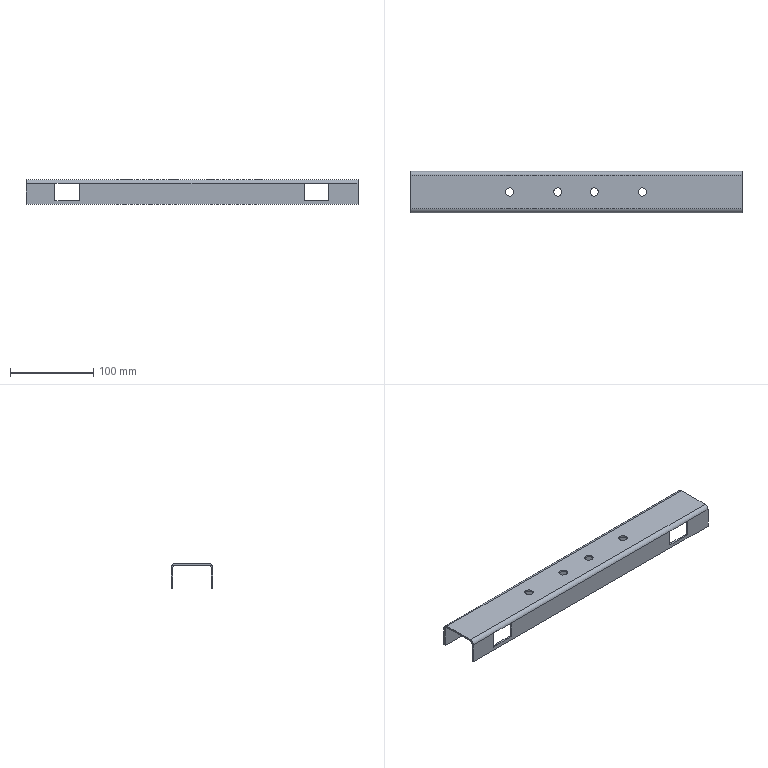Component | SolidWorks | 50x30x2ColdBentEqualAngleSteel400-1 | 1 solid | 52 faces | box 400 x 50 x 30 mm | volume 76567 mm3 | plane 34 | cylinder 18 | commonest cylinder face diameters 10 x10 6 x8
build123d program:
from build123d import *

# Parameters (mm, degrees)
BOSS_EXTRUDE1_DEPTH     = 400
SKETCH3_R               = 5
CUT_EXTRUDE1_2_DEPTH    = 65
SKETCH4_R               = 5
CUT_EXTRUDE2_DEPTH      = 65
CUT_EXTRUDE3_DEPTH      = 67
SKETCH6_W               = 30
SKETCH6_H               = 20
CUT_EXTRUDE4_DEPTH      = 67
FILLET1_R               = 3
CUT_EXTRUDE1_DEPTH      = 405.228
CUT_EXTRUDE1_DEPTH_BACK = 405.228
SKETCH1_W               = 5.72
SKETCH1_H               = 21


with BuildPart() as part:
    # Sketch1_2 → Boss-Extrude1 (new body)
    with BuildSketch(Plane(origin=(0, 0, 0), x_dir=(0, 0, -1), z_dir=(1, 0, 0))):
        with BuildLine():
            Line((0, 5), (0, 45))
            ThreePointArc((0, 45), (1.464, 48.536), (5, 50))
            Line((5, 50), (30, 50))
            Line((30, 50), (30, 48))
            Line((30, 48), (5, 48))
            ThreePointArc((5, 48), (2.879, 47.121), (2, 45))
            Line((2, 45), (2, 5))
            ThreePointArc((2, 5), (2.879, 2.879), (5, 2))
            Line((5, 2), (30, 2))
            Line((30, 2), (30, 0))
            Line((30, 0), (5, 0))
            ThreePointArc((5, 0), (1.464, 1.464), (0, 5))
        make_face()
    extrude(amount=BOSS_EXTRUDE1_DEPTH)

    # Sketch3 → Cut-Extrude1_2 (cut)
    with BuildSketch(Plane.XY):
        with Locations((120, 25)):
            Circle(SKETCH3_R)
        with Locations((280, 25)):
            Circle(SKETCH3_R)
    extrude(amount=-CUT_EXTRUDE1_2_DEPTH, mode=Mode.SUBTRACT)

    # Sketch4 → Cut-Extrude2 (cut)
    with BuildSketch(Plane.XY):
        with Locations((178, 25)):
            Circle(SKETCH4_R)
        with Locations((222, 25)):
            Circle(SKETCH4_R)
    extrude(amount=-CUT_EXTRUDE2_DEPTH, mode=Mode.SUBTRACT)

    # Sketch5 → Cut-Extrude3 (cut)
    with BuildSketch(Plane(origin=(0, 50, 0), x_dir=(1, 0, 0), z_dir=(0, 1, 0))):
        with BuildLine():
            Line((360, 25), (340, 25))
            ThreePointArc((340, 25), (336.464, 23.536), (335, 20))
            Line((335, 20), (335, 10))
            ThreePointArc((335, 10), (336.464, 6.464), (340, 5))
            Line((340, 5), (360, 5))
            ThreePointArc((360, 5), (363.536, 6.464), (365, 10))
            Line((365, 10), (365, 20))
            ThreePointArc((365, 20), (363.536, 23.536), (360, 25))
        make_face()
        with BuildLine():
            Line((65, 20), (65, 10))
            ThreePointArc((65, 10), (63.536, 6.464), (60, 5))
            Line((60, 5), (40, 5))
            ThreePointArc((40, 5), (36.464, 6.464), (35, 10))
            Line((35, 10), (35, 20))
            ThreePointArc((35, 20), (36.464, 23.536), (40, 25))
            Line((40, 25), (60, 25))
            ThreePointArc((60, 25), (63.536, 23.536), (65, 20))
        make_face()
    extrude(amount=-CUT_EXTRUDE3_DEPTH, mode=Mode.SUBTRACT)

    # Sketch6 → Cut-Extrude4 (cut)
    with BuildSketch(Plane(origin=(0, 50, 0), x_dir=(1, 0, 0), z_dir=(0, 1, 0))):
        with Locations((50, 15)):
            Rectangle(SKETCH6_W, SKETCH6_H)
        with Locations((350, 15)):
            Rectangle(SKETCH6_W, SKETCH6_H)
    extrude(amount=-CUT_EXTRUDE4_DEPTH, mode=Mode.SUBTRACT)

    # Fillet1
    fillet1_edges = [part.edges().sort_by_distance(p)[0] for p in [
        (65, 49, -5),
        (35, 49, -5),
        (65, 49, -25),
        (35, 49, -25),
        (365, 49, -25),
        (365, 49, -5),
        (335, 49, -5),
        (335, 49, -25),
    ]]
    fillet(fillet1_edges, radius=FILLET1_R)

    # Sketch1 → Cut-Extrude1 (cut, two sides: drawn at the far end of the back side and taken through both)
    with BuildSketch(Plane(origin=(0, 0, 0), x_dir=(1, 0, 0), z_dir=(0, 1, 0)).offset(-CUT_EXTRUDE1_DEPTH_BACK)):
        with Locations((37.14, 15)):
            Rectangle(SKETCH1_W, SKETCH1_H)
    extrude(amount=CUT_EXTRUDE1_DEPTH + CUT_EXTRUDE1_DEPTH_BACK, mode=Mode.SUBTRACT)


solid = part.part

# Placed as in the assembly
solid = solid.moved(Location((-174.371, 2.1, 415), (0, 0, 0)))